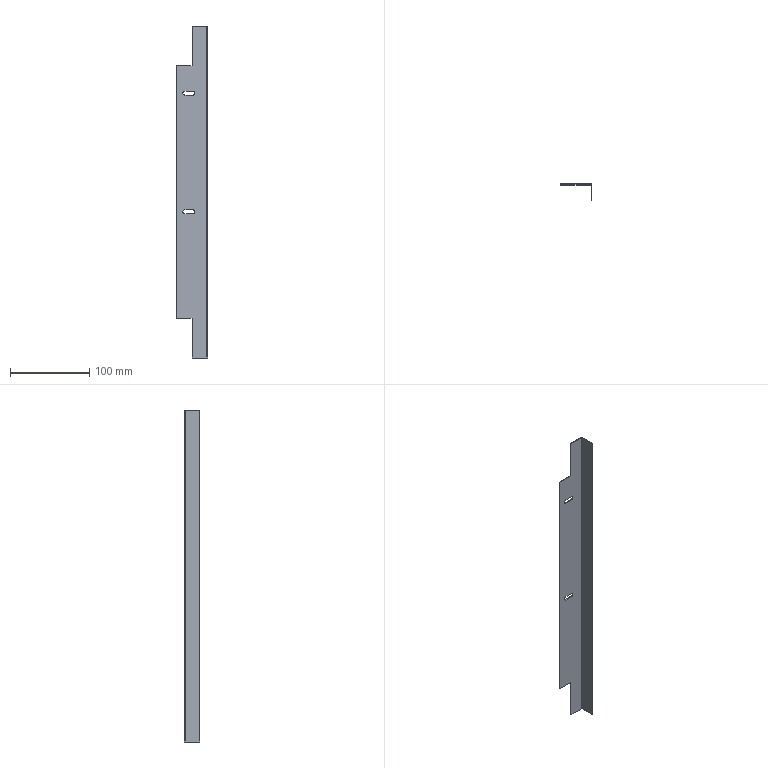Component | SolidWorks | CCQ-1.1-2UpperAngleIron-2 | 1 solid | 28 faces | box 40 x 20 x 420 mm | volume 22418 mm3 | plane 20 | cylinder 8 | commonest cylinder face diameters 5 x6 3.473 x1 1.473 x1 | material 304
STEP:
#1=COLOUR_RGB('',0.7922,0.8196,0.9333);
#2=FILL_AREA_STYLE_COLOUR('',#1);
#3=FILL_AREA_STYLE('',(#2));
#4=SURFACE_STYLE_FILL_AREA(#3);
#5=SURFACE_SIDE_STYLE('',(#4));
#6=SURFACE_STYLE_USAGE(.BOTH.,#5);
#7=PRESENTATION_STYLE_ASSIGNMENT((#6));
#8=CARTESIAN_POINT('',(0.2953,19.547,-8.819));
#9=VERTEX_POINT('',#8);
#10=CARTESIAN_POINT('',(0.3937,19.547,-8.72));
#11=VERTEX_POINT('',#10);
#12=CARTESIAN_POINT('',(0.3937,19.547,-8.819));
#13=DIRECTION('',(-0.,1.,0.));
#14=DIRECTION('',(-1.,0.,0.));
#15=AXIS2_PLACEMENT_3D('',#12,#13,#14);
#16=CIRCLE('',#15,0.09843);
#17=EDGE_CURVE('',#9,#11,#16,.T.);
#18=ORIENTED_EDGE('',*,*,#17,.F.);
#19=CARTESIAN_POINT('',(0.2953,19.587,-8.819));
#20=VERTEX_POINT('',#19);
#21=CARTESIAN_POINT('',(0.2953,19.193,-8.819));
#22=DIRECTION('',(-0.,1.,0.));
#23=VECTOR('',#22,39.37);
#24=LINE('',#21,#23);
#25=EDGE_CURVE('',#9,#20,#24,.T.);
#26=ORIENTED_EDGE('',*,*,#25,.T.);
#27=CARTESIAN_POINT('',(0.3937,19.587,-8.72));
#28=VERTEX_POINT('',#27);
#29=CARTESIAN_POINT('',(0.3937,19.587,-8.819));
#30=DIRECTION('',(-0.,1.,0.));
#31=DIRECTION('',(-1.,0.,0.));
#32=AXIS2_PLACEMENT_3D('',#29,#30,#31);
#33=CIRCLE('',#32,0.09843);
#34=EDGE_CURVE('',#20,#28,#33,.T.);
#35=ORIENTED_EDGE('',*,*,#34,.T.);
#36=CARTESIAN_POINT('',(0.3937,19.193,-8.72));
#37=DIRECTION('',(-0.,1.,0.));
#38=VECTOR('',#37,39.37);
#39=LINE('',#36,#38);
#40=EDGE_CURVE('',#11,#28,#39,.T.);
#41=ORIENTED_EDGE('',*,*,#40,.F.);
#42=EDGE_LOOP('',(#18,#26,#35,#41));
#43=FACE_OUTER_BOUND('',#42,.T.);
#44=CARTESIAN_POINT('',(0.3937,19.193,-8.819));
#45=DIRECTION('',(-0.,1.,0.));
#46=DIRECTION('',(-1.,0.,0.));
#47=AXIS2_PLACEMENT_3D('',#44,#45,#46);
#48=CYLINDRICAL_SURFACE('',#47,0.09843);
#49=ADVANCED_FACE('',(#43),#48,.F.);
#50=CARTESIAN_POINT('',(0.2953,19.547,-2.913));
#51=VERTEX_POINT('',#50);
#52=CARTESIAN_POINT('',(0.3937,19.547,-2.815));
#53=VERTEX_POINT('',#52);
#54=CARTESIAN_POINT('',(0.3937,19.547,-2.913));
#55=DIRECTION('',(-0.,1.,0.));
#56=DIRECTION('',(-1.,0.,0.));
#57=AXIS2_PLACEMENT_3D('',#54,#55,#56);
#58=CIRCLE('',#57,0.09843);
#59=EDGE_CURVE('',#51,#53,#58,.T.);
#60=ORIENTED_EDGE('',*,*,#59,.F.);
#61=CARTESIAN_POINT('',(0.2953,19.587,-2.913));
#62=VERTEX_POINT('',#61);
#63=CARTESIAN_POINT('',(0.2953,19.193,-2.913));
#64=DIRECTION('',(-0.,1.,0.));
#65=VECTOR('',#64,39.37);
#66=LINE('',#63,#65);
#67=EDGE_CURVE('',#51,#62,#66,.T.);
#68=ORIENTED_EDGE('',*,*,#67,.T.);
#69=CARTESIAN_POINT('',(0.3937,19.587,-2.815));
#70=VERTEX_POINT('',#69);
#71=CARTESIAN_POINT('',(0.3937,19.587,-2.913));
#72=DIRECTION('',(-0.,1.,0.));
#73=DIRECTION('',(-1.,0.,0.));
#74=AXIS2_PLACEMENT_3D('',#71,#72,#73);
#75=CIRCLE('',#74,0.09843);
#76=EDGE_CURVE('',#62,#70,#75,.T.);
#77=ORIENTED_EDGE('',*,*,#76,.T.);
#78=CARTESIAN_POINT('',(0.3937,19.193,-2.815));
#79=DIRECTION('',(-0.,1.,0.));
#80=VECTOR('',#79,39.37);
#81=LINE('',#78,#80);
#82=EDGE_CURVE('',#53,#70,#81,.T.);
#83=ORIENTED_EDGE('',*,*,#82,.F.);
#84=EDGE_LOOP('',(#60,#68,#77,#83));
#85=FACE_OUTER_BOUND('',#84,.T.);
#86=CARTESIAN_POINT('',(0.3937,19.193,-2.913));
#87=DIRECTION('',(-0.,1.,0.));
#88=DIRECTION('',(-1.,0.,0.));
#89=AXIS2_PLACEMENT_3D('',#86,#87,#88);
#90=CYLINDRICAL_SURFACE('',#89,0.09843);
#91=ADVANCED_FACE('',(#85),#90,.F.);
#92=CARTESIAN_POINT('',(1.535,19.518,0.4331));
#93=VERTEX_POINT('',#92);
#94=CARTESIAN_POINT('',(1.496,19.518,0.4331));
#95=VERTEX_POINT('',#94);
#96=CARTESIAN_POINT('',(1.535,19.518,0.4331));
#97=DIRECTION('',(-1.,-0.,0.));
#98=VECTOR('',#97,39.37);
#99=LINE('',#96,#98);
#100=EDGE_CURVE('',#93,#95,#99,.T.);
#101=ORIENTED_EDGE('',*,*,#100,.F.);
#102=CARTESIAN_POINT('',(1.467,19.587,0.4331));
#103=VERTEX_POINT('',#102);
#104=CARTESIAN_POINT('',(1.467,19.518,0.4331));
#105=DIRECTION('',(-0.,0.,-1.));
#106=DIRECTION('',(1.,0.,0.));
#107=AXIS2_PLACEMENT_3D('',#104,#105,#106);
#108=CIRCLE('',#107,0.06837);
#109=EDGE_CURVE('',#103,#93,#108,.T.);
#110=ORIENTED_EDGE('',*,*,#109,.F.);
#111=CARTESIAN_POINT('',(1.467,19.547,0.4331));
#112=VERTEX_POINT('',#111);
#113=CARTESIAN_POINT('',(1.467,19.547,0.4331));
#114=DIRECTION('',(0.,1.,0.));
#115=VECTOR('',#114,39.37);
#116=LINE('',#113,#115);
#117=EDGE_CURVE('',#112,#103,#116,.T.);
#118=ORIENTED_EDGE('',*,*,#117,.F.);
#119=CARTESIAN_POINT('',(1.467,19.518,0.4331));
#120=DIRECTION('',(-0.,0.,-1.));
#121=DIRECTION('',(1.,0.,0.));
#122=AXIS2_PLACEMENT_3D('',#119,#120,#121);
#123=CIRCLE('',#122,0.029);
#124=EDGE_CURVE('',#112,#95,#123,.T.);
#125=ORIENTED_EDGE('',*,*,#124,.T.);
#126=EDGE_LOOP('',(#101,#110,#118,#125));
#127=FACE_OUTER_BOUND('',#126,.T.);
#128=CARTESIAN_POINT('',(1.535,19.518,0.4331));
#129=DIRECTION('',(0.,-0.,1.));
#130=DIRECTION('',(1.,0.,-0.));
#131=AXIS2_PLACEMENT_3D('',#128,#129,#130);
#132=PLANE('',#131);
#133=ADVANCED_FACE('',(#127),#132,.T.);
#134=CARTESIAN_POINT('',(1.535,18.799,0.4331));
#135=VERTEX_POINT('',#134);
#136=CARTESIAN_POINT('',(1.535,19.587,0.4331));
#137=DIRECTION('',(0.,-1.,-0.));
#138=VECTOR('',#137,39.37);
#139=LINE('',#136,#138);
#140=EDGE_CURVE('',#93,#135,#139,.T.);
#141=ORIENTED_EDGE('',*,*,#140,.F.);
#142=ORIENTED_EDGE('',*,*,#100,.T.);
#143=CARTESIAN_POINT('',(1.496,18.799,0.4331));
#144=VERTEX_POINT('',#143);
#145=CARTESIAN_POINT('',(1.496,19.587,0.4331));
#146=DIRECTION('',(0.,-1.,-0.));
#147=VECTOR('',#146,39.37);
#148=LINE('',#145,#147);
#149=EDGE_CURVE('',#95,#144,#148,.T.);
#150=ORIENTED_EDGE('',*,*,#149,.T.);
#151=CARTESIAN_POINT('',(1.535,18.799,0.4331));
#152=DIRECTION('',(-1.,-0.,0.));
#153=VECTOR('',#152,39.37);
#154=LINE('',#151,#153);
#155=EDGE_CURVE('',#135,#144,#154,.T.);
#156=ORIENTED_EDGE('',*,*,#155,.F.);
#157=EDGE_LOOP('',(#141,#142,#150,#156));
#158=FACE_OUTER_BOUND('',#157,.T.);
#159=CARTESIAN_POINT('',(1.467,19.547,0.4331));
#160=DIRECTION('',(0.,-0.,1.));
#161=DIRECTION('',(1.,0.,-0.));
#162=AXIS2_PLACEMENT_3D('',#159,#160,#161);
#163=PLANE('',#162);
#164=ADVANCED_FACE('',(#158),#163,.T.);
#165=CARTESIAN_POINT('',(1.467,19.587,-16.102));
#166=VERTEX_POINT('',#165);
#167=CARTESIAN_POINT('',(1.467,19.547,-16.102));
#168=VERTEX_POINT('',#167);
#169=CARTESIAN_POINT('',(1.467,19.587,-16.102));
#170=DIRECTION('',(-0.,-1.,-0.));
#171=VECTOR('',#170,39.37);
#172=LINE('',#169,#171);
#173=EDGE_CURVE('',#166,#168,#172,.T.);
#174=ORIENTED_EDGE('',*,*,#173,.F.);
#175=CARTESIAN_POINT('',(1.535,19.518,-16.102));
#176=VERTEX_POINT('',#175);
#177=CARTESIAN_POINT('',(1.467,19.518,-16.102));
#178=DIRECTION('',(-0.,0.,-1.));
#179=DIRECTION('',(1.,0.,0.));
#180=AXIS2_PLACEMENT_3D('',#177,#178,#179);
#181=CIRCLE('',#180,0.06837);
#182=EDGE_CURVE('',#166,#176,#181,.T.);
#183=ORIENTED_EDGE('',*,*,#182,.T.);
#184=CARTESIAN_POINT('',(1.496,19.518,-16.102));
#185=VERTEX_POINT('',#184);
#186=CARTESIAN_POINT('',(1.496,19.518,-16.102));
#187=DIRECTION('',(1.,0.,-0.));
#188=VECTOR('',#187,39.37);
#189=LINE('',#186,#188);
#190=EDGE_CURVE('',#185,#176,#189,.T.);
#191=ORIENTED_EDGE('',*,*,#190,.F.);
#192=CARTESIAN_POINT('',(1.467,19.518,-16.102));
#193=DIRECTION('',(-0.,0.,-1.));
#194=DIRECTION('',(1.,0.,0.));
#195=AXIS2_PLACEMENT_3D('',#192,#193,#194);
#196=CIRCLE('',#195,0.029);
#197=EDGE_CURVE('',#168,#185,#196,.T.);
#198=ORIENTED_EDGE('',*,*,#197,.F.);
#199=EDGE_LOOP('',(#174,#183,#191,#198));
#200=FACE_OUTER_BOUND('',#199,.T.);
#201=CARTESIAN_POINT('',(1.467,19.587,-16.102));
#202=DIRECTION('',(-0.,0.,-1.));
#203=DIRECTION('',(-1.,-0.,0.));
#204=AXIS2_PLACEMENT_3D('',#201,#202,#203);
#205=PLANE('',#204);
#206=ADVANCED_FACE('',(#200),#205,.T.);
#207=CARTESIAN_POINT('',(0.748,19.547,-16.102));
#208=VERTEX_POINT('',#207);
#209=CARTESIAN_POINT('',(0.748,19.587,-16.102));
#210=VERTEX_POINT('',#209);
#211=CARTESIAN_POINT('',(0.748,19.193,-16.102));
#212=DIRECTION('',(-0.,1.,0.));
#213=VECTOR('',#212,39.37);
#214=LINE('',#211,#213);
#215=EDGE_CURVE('',#208,#210,#214,.T.);
#216=ORIENTED_EDGE('',*,*,#215,.T.);
#217=CARTESIAN_POINT('',(-0.03937,19.587,-16.102));
#218=DIRECTION('',(1.,0.,-0.));
#219=VECTOR('',#218,39.37);
#220=LINE('',#217,#219);
#221=EDGE_CURVE('',#210,#166,#220,.T.);
#222=ORIENTED_EDGE('',*,*,#221,.T.);
#223=ORIENTED_EDGE('',*,*,#173,.T.);
#224=CARTESIAN_POINT('',(-0.03937,19.547,-16.102));
#225=DIRECTION('',(1.,0.,-0.));
#226=VECTOR('',#225,39.37);
#227=LINE('',#224,#226);
#228=EDGE_CURVE('',#208,#168,#227,.T.);
#229=ORIENTED_EDGE('',*,*,#228,.F.);
#230=EDGE_LOOP('',(#216,#222,#223,#229));
#231=FACE_OUTER_BOUND('',#230,.T.);
#232=CARTESIAN_POINT('',(1.496,19.518,-16.102));
#233=DIRECTION('',(-0.,0.,-1.));
#234=DIRECTION('',(-1.,-0.,0.));
#235=AXIS2_PLACEMENT_3D('',#232,#233,#234);
#236=PLANE('',#235);
#237=ADVANCED_FACE('',(#231),#236,.T.);
#238=CARTESIAN_POINT('',(1.496,18.799,-16.102));
#239=VERTEX_POINT('',#238);
#240=CARTESIAN_POINT('',(1.496,19.587,-16.102));
#241=DIRECTION('',(0.,-1.,-0.));
#242=VECTOR('',#241,39.37);
#243=LINE('',#240,#242);
#244=EDGE_CURVE('',#185,#239,#243,.T.);
#245=ORIENTED_EDGE('',*,*,#244,.T.);
#246=CARTESIAN_POINT('',(1.496,18.799,0.4331));
#247=DIRECTION('',(-0.,0.,-1.));
#248=VECTOR('',#247,39.37);
#249=LINE('',#246,#248);
#250=EDGE_CURVE('',#144,#239,#249,.T.);
#251=ORIENTED_EDGE('',*,*,#250,.F.);
#252=ORIENTED_EDGE('',*,*,#149,.F.);
#253=CARTESIAN_POINT('',(1.496,19.518,0.4331));
#254=DIRECTION('',(-0.,0.,-1.));
#255=VECTOR('',#254,39.37);
#256=LINE('',#253,#255);
#257=EDGE_CURVE('',#95,#185,#256,.T.);
#258=ORIENTED_EDGE('',*,*,#257,.T.);
#259=EDGE_LOOP('',(#245,#251,#252,#258));
#260=FACE_OUTER_BOUND('',#259,.T.);
#261=CARTESIAN_POINT('',(1.496,19.587,0.4331));
#262=DIRECTION('',(1.,0.,-0.));
#263=DIRECTION('',(-0.,0.,-1.));
#264=AXIS2_PLACEMENT_3D('',#261,#262,#263);
#265=PLANE('',#264);
#266=ADVANCED_FACE('',(#260),#265,.F.);
#267=CARTESIAN_POINT('',(1.535,18.799,-16.102));
#268=VERTEX_POINT('',#267);
#269=CARTESIAN_POINT('',(1.535,18.799,-16.102));
#270=DIRECTION('',(-1.,-0.,0.));
#271=VECTOR('',#270,39.37);
#272=LINE('',#269,#271);
#273=EDGE_CURVE('',#268,#239,#272,.T.);
#274=ORIENTED_EDGE('',*,*,#273,.F.);
#275=CARTESIAN_POINT('',(1.535,18.799,0.4331));
#276=DIRECTION('',(-0.,0.,-1.));
#277=VECTOR('',#276,39.37);
#278=LINE('',#275,#277);
#279=EDGE_CURVE('',#135,#268,#278,.T.);
#280=ORIENTED_EDGE('',*,*,#279,.F.);
#281=ORIENTED_EDGE('',*,*,#155,.T.);
#282=ORIENTED_EDGE('',*,*,#250,.T.);
#283=EDGE_LOOP('',(#274,#280,#281,#282));
#284=FACE_OUTER_BOUND('',#283,.T.);
#285=CARTESIAN_POINT('',(1.535,18.799,0.4331));
#286=DIRECTION('',(0.,-1.,-0.));
#287=DIRECTION('',(1.,0.,-0.));
#288=AXIS2_PLACEMENT_3D('',#285,#286,#287);
#289=PLANE('',#288);
#290=ADVANCED_FACE('',(#284),#289,.T.);
#291=CARTESIAN_POINT('',(1.535,19.587,-16.102));
#292=DIRECTION('',(0.,-1.,-0.));
#293=VECTOR('',#292,39.37);
#294=LINE('',#291,#293);
#295=EDGE_CURVE('',#176,#268,#294,.T.);
#296=ORIENTED_EDGE('',*,*,#295,.F.);
#297=CARTESIAN_POINT('',(1.535,19.518,0.4331));
#298=DIRECTION('',(-0.,0.,-1.));
#299=VECTOR('',#298,39.37);
#300=LINE('',#297,#299);
#301=EDGE_CURVE('',#93,#176,#300,.T.);
#302=ORIENTED_EDGE('',*,*,#301,.F.);
#303=ORIENTED_EDGE('',*,*,#140,.T.);
#304=ORIENTED_EDGE('',*,*,#279,.T.);
#305=EDGE_LOOP('',(#296,#302,#303,#304));
#306=FACE_OUTER_BOUND('',#305,.T.);
#307=CARTESIAN_POINT('',(1.535,19.587,0.4331));
#308=DIRECTION('',(1.,0.,-0.));
#309=DIRECTION('',(-0.,0.,-1.));
#310=AXIS2_PLACEMENT_3D('',#307,#308,#309);
#311=PLANE('',#310);
#312=ADVANCED_FACE('',(#306),#311,.T.);
#313=ORIENTED_EDGE('',*,*,#182,.F.);
#314=CARTESIAN_POINT('',(1.467,19.587,0.4331));
#315=DIRECTION('',(-0.,0.,-1.));
#316=VECTOR('',#315,39.37);
#317=LINE('',#314,#316);
#318=EDGE_CURVE('',#103,#166,#317,.T.);
#319=ORIENTED_EDGE('',*,*,#318,.F.);
#320=ORIENTED_EDGE('',*,*,#109,.T.);
#321=ORIENTED_EDGE('',*,*,#301,.T.);
#322=EDGE_LOOP('',(#313,#319,#320,#321));
#323=FACE_OUTER_BOUND('',#322,.T.);
#324=CARTESIAN_POINT('',(1.467,19.518,0.4331));
#325=DIRECTION('',(-0.,0.,-1.));
#326=DIRECTION('',(-1.,0.,0.));
#327=AXIS2_PLACEMENT_3D('',#324,#325,#326);
#328=CYLINDRICAL_SURFACE('',#327,0.06837);
#329=ADVANCED_FACE('',(#323),#328,.T.);
#330=CARTESIAN_POINT('',(0.7874,19.587,-8.72));
#331=VERTEX_POINT('',#330);
#332=CARTESIAN_POINT('',(0.7874,19.587,-8.917));
#333=VERTEX_POINT('',#332);
#334=CARTESIAN_POINT('',(0.7874,19.587,-8.819));
#335=DIRECTION('',(-0.,1.,0.));
#336=DIRECTION('',(-1.,0.,0.));
#337=AXIS2_PLACEMENT_3D('',#334,#335,#336);
#338=CIRCLE('',#337,0.09843);
#339=EDGE_CURVE('',#331,#333,#338,.T.);
#340=ORIENTED_EDGE('',*,*,#339,.F.);
#341=CARTESIAN_POINT('',(0.7874,19.587,-8.72));
#342=DIRECTION('',(1.,0.,-0.));
#343=VECTOR('',#342,39.37);
#344=LINE('',#341,#343);
#345=EDGE_CURVE('',#28,#331,#344,.T.);
#346=ORIENTED_EDGE('',*,*,#345,.F.);
#347=ORIENTED_EDGE('',*,*,#34,.F.);
#348=CARTESIAN_POINT('',(0.3937,19.587,-8.917));
#349=VERTEX_POINT('',#348);
#350=CARTESIAN_POINT('',(0.3937,19.587,-8.819));
#351=DIRECTION('',(-0.,1.,0.));
#352=DIRECTION('',(-1.,0.,0.));
#353=AXIS2_PLACEMENT_3D('',#350,#351,#352);
#354=CIRCLE('',#353,0.09843);
#355=EDGE_CURVE('',#349,#20,#354,.T.);
#356=ORIENTED_EDGE('',*,*,#355,.F.);
#357=CARTESIAN_POINT('',(0.7874,19.587,-8.917));
#358=DIRECTION('',(-1.,-0.,0.));
#359=VECTOR('',#358,39.37);
#360=LINE('',#357,#359);
#361=EDGE_CURVE('',#333,#349,#360,.T.);
#362=ORIENTED_EDGE('',*,*,#361,.F.);
#363=EDGE_LOOP('',(#340,#346,#347,#356,#362));
#364=FACE_BOUND('',#363,.T.);
#365=CARTESIAN_POINT('',(0.7874,19.587,-2.815));
#366=VERTEX_POINT('',#365);
#367=CARTESIAN_POINT('',(0.7874,19.587,-3.012));
#368=VERTEX_POINT('',#367);
#369=CARTESIAN_POINT('',(0.7874,19.587,-2.913));
#370=DIRECTION('',(-0.,1.,0.));
#371=DIRECTION('',(-1.,0.,0.));
#372=AXIS2_PLACEMENT_3D('',#369,#370,#371);
#373=CIRCLE('',#372,0.09843);
#374=EDGE_CURVE('',#366,#368,#373,.T.);
#375=ORIENTED_EDGE('',*,*,#374,.F.);
#376=CARTESIAN_POINT('',(0.7874,19.587,-2.815));
#377=DIRECTION('',(1.,0.,-0.));
#378=VECTOR('',#377,39.37);
#379=LINE('',#376,#378);
#380=EDGE_CURVE('',#70,#366,#379,.T.);
#381=ORIENTED_EDGE('',*,*,#380,.F.);
#382=ORIENTED_EDGE('',*,*,#76,.F.);
#383=CARTESIAN_POINT('',(0.3937,19.587,-3.012));
#384=VERTEX_POINT('',#383);
#385=CARTESIAN_POINT('',(0.3937,19.587,-2.913));
#386=DIRECTION('',(-0.,1.,0.));
#387=DIRECTION('',(-1.,0.,0.));
#388=AXIS2_PLACEMENT_3D('',#385,#386,#387);
#389=CIRCLE('',#388,0.09843);
#390=EDGE_CURVE('',#384,#62,#389,.T.);
#391=ORIENTED_EDGE('',*,*,#390,.F.);
#392=CARTESIAN_POINT('',(0.7874,19.587,-3.012));
#393=DIRECTION('',(-1.,-0.,0.));
#394=VECTOR('',#393,39.37);
#395=LINE('',#392,#394);
#396=EDGE_CURVE('',#368,#384,#395,.T.);
#397=ORIENTED_EDGE('',*,*,#396,.F.);
#398=EDGE_LOOP('',(#375,#381,#382,#391,#397));
#399=FACE_BOUND('',#398,.T.);
#400=CARTESIAN_POINT('',(0.748,19.587,0.4331));
#401=VERTEX_POINT('',#400);
#402=CARTESIAN_POINT('',(0.748,19.587,-1.535));
#403=VERTEX_POINT('',#402);
#404=CARTESIAN_POINT('',(0.748,19.587,0.4331));
#405=DIRECTION('',(-0.,0.,-1.));
#406=VECTOR('',#405,39.37);
#407=LINE('',#404,#406);
#408=EDGE_CURVE('',#401,#403,#407,.T.);
#409=ORIENTED_EDGE('',*,*,#408,.F.);
#410=CARTESIAN_POINT('',(-0.03937,19.587,0.4331));
#411=DIRECTION('',(1.,0.,-0.));
#412=VECTOR('',#411,39.37);
#413=LINE('',#410,#412);
#414=EDGE_CURVE('',#401,#103,#413,.T.);
#415=ORIENTED_EDGE('',*,*,#414,.T.);
#416=ORIENTED_EDGE('',*,*,#318,.T.);
#417=ORIENTED_EDGE('',*,*,#221,.F.);
#418=CARTESIAN_POINT('',(0.748,19.587,-14.134));
#419=VERTEX_POINT('',#418);
#420=CARTESIAN_POINT('',(0.748,19.587,-16.102));
#421=DIRECTION('',(-0.,0.,-1.));
#422=VECTOR('',#421,39.37);
#423=LINE('',#420,#422);
#424=EDGE_CURVE('',#419,#210,#423,.T.);
#425=ORIENTED_EDGE('',*,*,#424,.F.);
#426=CARTESIAN_POINT('',(-0.03937,19.587,-14.134));
#427=VERTEX_POINT('',#426);
#428=CARTESIAN_POINT('',(0.748,19.587,-14.134));
#429=DIRECTION('',(1.,0.,-0.));
#430=VECTOR('',#429,39.37);
#431=LINE('',#428,#430);
#432=EDGE_CURVE('',#427,#419,#431,.T.);
#433=ORIENTED_EDGE('',*,*,#432,.F.);
#434=CARTESIAN_POINT('',(-0.03937,19.587,-1.535));
#435=VERTEX_POINT('',#434);
#436=CARTESIAN_POINT('',(-0.03937,19.587,0.4331));
#437=DIRECTION('',(-0.,0.,-1.));
#438=VECTOR('',#437,39.37);
#439=LINE('',#436,#438);
#440=EDGE_CURVE('',#435,#427,#439,.T.);
#441=ORIENTED_EDGE('',*,*,#440,.F.);
#442=CARTESIAN_POINT('',(0.748,19.587,-1.535));
#443=DIRECTION('',(-1.,-0.,0.));
#444=VECTOR('',#443,39.37);
#445=LINE('',#442,#444);
#446=EDGE_CURVE('',#403,#435,#445,.T.);
#447=ORIENTED_EDGE('',*,*,#446,.F.);
#448=EDGE_LOOP('',(#409,#415,#416,#417,#425,#433,#441,#447));
#449=FACE_OUTER_BOUND('',#448,.T.);
#450=CARTESIAN_POINT('',(-0.03937,19.587,0.4331));
#451=DIRECTION('',(-0.,1.,0.));
#452=DIRECTION('',(-1.,-0.,0.));
#453=AXIS2_PLACEMENT_3D('',#450,#451,#452);
#454=PLANE('',#453);
#455=ADVANCED_FACE('',(#364,#399,#449),#454,.T.);
#456=CARTESIAN_POINT('',(-0.03937,19.547,-1.535));
#457=VERTEX_POINT('',#456);
#458=CARTESIAN_POINT('',(-0.03937,19.193,-1.535));
#459=DIRECTION('',(-0.,1.,0.));
#460=VECTOR('',#459,39.37);
#461=LINE('',#458,#460);
#462=EDGE_CURVE('',#457,#435,#461,.T.);
#463=ORIENTED_EDGE('',*,*,#462,.T.);
#464=ORIENTED_EDGE('',*,*,#440,.T.);
#465=CARTESIAN_POINT('',(-0.03937,19.547,-14.134));
#466=VERTEX_POINT('',#465);
#467=CARTESIAN_POINT('',(-0.03937,19.193,-14.134));
#468=DIRECTION('',(-0.,1.,0.));
#469=VECTOR('',#468,39.37);
#470=LINE('',#467,#469);
#471=EDGE_CURVE('',#466,#427,#470,.T.);
#472=ORIENTED_EDGE('',*,*,#471,.F.);
#473=CARTESIAN_POINT('',(-0.03937,19.547,0.4331));
#474=DIRECTION('',(-0.,0.,-1.));
#475=VECTOR('',#474,39.37);
#476=LINE('',#473,#475);
#477=EDGE_CURVE('',#457,#466,#476,.T.);
#478=ORIENTED_EDGE('',*,*,#477,.F.);
#479=EDGE_LOOP('',(#463,#464,#472,#478));
#480=FACE_OUTER_BOUND('',#479,.T.);
#481=CARTESIAN_POINT('',(-0.03937,19.547,0.4331));
#482=DIRECTION('',(-1.,-0.,0.));
#483=DIRECTION('',(0.,-0.,1.));
#484=AXIS2_PLACEMENT_3D('',#481,#482,#483);
#485=PLANE('',#484);
#486=ADVANCED_FACE('',(#480),#485,.T.);
#487=CARTESIAN_POINT('',(0.7874,19.547,-8.72));
#488=VERTEX_POINT('',#487);
#489=CARTESIAN_POINT('',(-0.03937,19.547,-8.72));
#490=DIRECTION('',(1.,0.,-0.));
#491=VECTOR('',#490,39.37);
#492=LINE('',#489,#491);
#493=EDGE_CURVE('',#11,#488,#492,.T.);
#494=ORIENTED_EDGE('',*,*,#493,.T.);
#495=CARTESIAN_POINT('',(0.7874,19.547,-8.917));
#496=VERTEX_POINT('',#495);
#497=CARTESIAN_POINT('',(0.7874,19.547,-8.819));
#498=DIRECTION('',(-0.,1.,0.));
#499=DIRECTION('',(-1.,0.,0.));
#500=AXIS2_PLACEMENT_3D('',#497,#498,#499);
#501=CIRCLE('',#500,0.09843);
#502=EDGE_CURVE('',#488,#496,#501,.T.);
#503=ORIENTED_EDGE('',*,*,#502,.T.);
#504=CARTESIAN_POINT('',(0.3937,19.547,-8.917));
#505=VERTEX_POINT('',#504);
#506=CARTESIAN_POINT('',(-0.03937,19.547,-8.917));
#507=DIRECTION('',(-1.,-0.,0.));
#508=VECTOR('',#507,39.37);
#509=LINE('',#506,#508);
#510=EDGE_CURVE('',#496,#505,#509,.T.);
#511=ORIENTED_EDGE('',*,*,#510,.T.);
#512=CARTESIAN_POINT('',(0.3937,19.547,-8.819));
#513=DIRECTION('',(-0.,1.,0.));
#514=DIRECTION('',(-1.,0.,0.));
#515=AXIS2_PLACEMENT_3D('',#512,#513,#514);
#516=CIRCLE('',#515,0.09843);
#517=EDGE_CURVE('',#505,#9,#516,.T.);
#518=ORIENTED_EDGE('',*,*,#517,.T.);
#519=ORIENTED_EDGE('',*,*,#17,.T.);
#520=EDGE_LOOP('',(#494,#503,#511,#518,#519));
#521=FACE_BOUND('',#520,.T.);
#522=CARTESIAN_POINT('',(0.7874,19.547,-2.815));
#523=VERTEX_POINT('',#522);
#524=CARTESIAN_POINT('',(-0.03937,19.547,-2.815));
#525=DIRECTION('',(1.,0.,-0.));
#526=VECTOR('',#525,39.37);
#527=LINE('',#524,#526);
#528=EDGE_CURVE('',#53,#523,#527,.T.);
#529=ORIENTED_EDGE('',*,*,#528,.T.);
#530=CARTESIAN_POINT('',(0.7874,19.547,-3.012));
#531=VERTEX_POINT('',#530);
#532=CARTESIAN_POINT('',(0.7874,19.547,-2.913));
#533=DIRECTION('',(-0.,1.,0.));
#534=DIRECTION('',(-1.,0.,0.));
#535=AXIS2_PLACEMENT_3D('',#532,#533,#534);
#536=CIRCLE('',#535,0.09843);
#537=EDGE_CURVE('',#523,#531,#536,.T.);
#538=ORIENTED_EDGE('',*,*,#537,.T.);
#539=CARTESIAN_POINT('',(0.3937,19.547,-3.012));
#540=VERTEX_POINT('',#539);
#541=CARTESIAN_POINT('',(-0.03937,19.547,-3.012));
#542=DIRECTION('',(-1.,-0.,0.));
#543=VECTOR('',#542,39.37);
#544=LINE('',#541,#543);
#545=EDGE_CURVE('',#531,#540,#544,.T.);
#546=ORIENTED_EDGE('',*,*,#545,.T.);
#547=CARTESIAN_POINT('',(0.3937,19.547,-2.913));
#548=DIRECTION('',(-0.,1.,0.));
#549=DIRECTION('',(-1.,0.,0.));
#550=AXIS2_PLACEMENT_3D('',#547,#548,#549);
#551=CIRCLE('',#550,0.09843);
#552=EDGE_CURVE('',#540,#51,#551,.T.);
#553=ORIENTED_EDGE('',*,*,#552,.T.);
#554=ORIENTED_EDGE('',*,*,#59,.T.);
#555=EDGE_LOOP('',(#529,#538,#546,#553,#554));
#556=FACE_BOUND('',#555,.T.);
#557=CARTESIAN_POINT('',(0.748,19.547,0.4331));
#558=VERTEX_POINT('',#557);
#559=CARTESIAN_POINT('',(-0.03937,19.547,0.4331));
#560=DIRECTION('',(1.,0.,-0.));
#561=VECTOR('',#560,39.37);
#562=LINE('',#559,#561);
#563=EDGE_CURVE('',#558,#112,#562,.T.);
#564=ORIENTED_EDGE('',*,*,#563,.F.);
#565=CARTESIAN_POINT('',(0.748,19.547,-1.535));
#566=VERTEX_POINT('',#565);
#567=CARTESIAN_POINT('',(0.748,19.547,0.4331));
#568=DIRECTION('',(-0.,0.,-1.));
#569=VECTOR('',#568,39.37);
#570=LINE('',#567,#569);
#571=EDGE_CURVE('',#558,#566,#570,.T.);
#572=ORIENTED_EDGE('',*,*,#571,.T.);
#573=CARTESIAN_POINT('',(-0.03937,19.547,-1.535));
#574=DIRECTION('',(-1.,-0.,0.));
#575=VECTOR('',#574,39.37);
#576=LINE('',#573,#575);
#577=EDGE_CURVE('',#566,#457,#576,.T.);
#578=ORIENTED_EDGE('',*,*,#577,.T.);
#579=ORIENTED_EDGE('',*,*,#477,.T.);
#580=CARTESIAN_POINT('',(0.748,19.547,-14.134));
#581=VERTEX_POINT('',#580);
#582=CARTESIAN_POINT('',(-0.03937,19.547,-14.134));
#583=DIRECTION('',(1.,0.,-0.));
#584=VECTOR('',#583,39.37);
#585=LINE('',#582,#584);
#586=EDGE_CURVE('',#466,#581,#585,.T.);
#587=ORIENTED_EDGE('',*,*,#586,.T.);
#588=CARTESIAN_POINT('',(0.748,19.547,0.4331));
#589=DIRECTION('',(-0.,0.,-1.));
#590=VECTOR('',#589,39.37);
#591=LINE('',#588,#590);
#592=EDGE_CURVE('',#581,#208,#591,.T.);
#593=ORIENTED_EDGE('',*,*,#592,.T.);
#594=ORIENTED_EDGE('',*,*,#228,.T.);
#595=CARTESIAN_POINT('',(1.467,19.547,0.4331));
#596=DIRECTION('',(-0.,0.,-1.));
#597=VECTOR('',#596,39.37);
#598=LINE('',#595,#597);
#599=EDGE_CURVE('',#112,#168,#598,.T.);
#600=ORIENTED_EDGE('',*,*,#599,.F.);
#601=EDGE_LOOP('',(#564,#572,#578,#579,#587,#593,#594,#600));
#602=FACE_OUTER_BOUND('',#601,.T.);
#603=CARTESIAN_POINT('',(-0.03937,19.547,0.4331));
#604=DIRECTION('',(-0.,1.,0.));
#605=DIRECTION('',(-1.,-0.,0.));
#606=AXIS2_PLACEMENT_3D('',#603,#604,#605);
#607=PLANE('',#606);
#608=ADVANCED_FACE('',(#521,#556,#602),#607,.F.);
#609=ORIENTED_EDGE('',*,*,#197,.T.);
#610=ORIENTED_EDGE('',*,*,#257,.F.);
#611=ORIENTED_EDGE('',*,*,#124,.F.);
#612=ORIENTED_EDGE('',*,*,#599,.T.);
#613=EDGE_LOOP('',(#609,#610,#611,#612));
#614=FACE_OUTER_BOUND('',#613,.T.);
#615=CARTESIAN_POINT('',(1.467,19.518,0.4331));
#616=DIRECTION('',(-0.,0.,-1.));
#617=DIRECTION('',(-1.,0.,0.));
#618=AXIS2_PLACEMENT_3D('',#615,#616,#617);
#619=CYLINDRICAL_SURFACE('',#618,0.029);
#620=ADVANCED_FACE('',(#614),#619,.F.);
#621=CARTESIAN_POINT('',(0.748,19.518,0.4331));
#622=DIRECTION('',(-0.,1.,0.));
#623=VECTOR('',#622,39.37);
#624=LINE('',#621,#623);
#625=EDGE_CURVE('',#558,#401,#624,.T.);
#626=ORIENTED_EDGE('',*,*,#625,.F.);
#627=ORIENTED_EDGE('',*,*,#563,.T.);
#628=ORIENTED_EDGE('',*,*,#117,.T.);
#629=ORIENTED_EDGE('',*,*,#414,.F.);
#630=EDGE_LOOP('',(#626,#627,#628,#629));
#631=FACE_OUTER_BOUND('',#630,.T.);
#632=CARTESIAN_POINT('',(1.467,19.518,0.4331));
#633=DIRECTION('',(0.,-0.,1.));
#634=DIRECTION('',(1.,0.,-0.));
#635=AXIS2_PLACEMENT_3D('',#632,#633,#634);
#636=PLANE('',#635);
#637=ADVANCED_FACE('',(#631),#636,.T.);
#638=ORIENTED_EDGE('',*,*,#244,.F.);
#639=ORIENTED_EDGE('',*,*,#190,.T.);
#640=ORIENTED_EDGE('',*,*,#295,.T.);
#641=ORIENTED_EDGE('',*,*,#273,.T.);
#642=EDGE_LOOP('',(#638,#639,#640,#641));
#643=FACE_OUTER_BOUND('',#642,.T.);
#644=CARTESIAN_POINT('',(1.467,19.518,-16.102));
#645=DIRECTION('',(0.,-0.,1.));
#646=DIRECTION('',(1.,0.,-0.));
#647=AXIS2_PLACEMENT_3D('',#644,#645,#646);
#648=PLANE('',#647);
#649=ADVANCED_FACE('',(#643),#648,.F.);
#650=CARTESIAN_POINT('',(0.748,19.193,-14.134));
#651=DIRECTION('',(-0.,1.,0.));
#652=VECTOR('',#651,39.37);
#653=LINE('',#650,#652);
#654=EDGE_CURVE('',#581,#419,#653,.T.);
#655=ORIENTED_EDGE('',*,*,#654,.T.);
#656=ORIENTED_EDGE('',*,*,#424,.T.);
#657=ORIENTED_EDGE('',*,*,#215,.F.);
#658=ORIENTED_EDGE('',*,*,#592,.F.);
#659=EDGE_LOOP('',(#655,#656,#657,#658));
#660=FACE_OUTER_BOUND('',#659,.T.);
#661=CARTESIAN_POINT('',(0.748,19.193,-16.102));
#662=DIRECTION('',(1.,0.,-0.));
#663=DIRECTION('',(-0.,0.,-1.));
#664=AXIS2_PLACEMENT_3D('',#661,#662,#663);
#665=PLANE('',#664);
#666=ADVANCED_FACE('',(#660),#665,.F.);
#667=ORIENTED_EDGE('',*,*,#471,.T.);
#668=ORIENTED_EDGE('',*,*,#432,.T.);
#669=ORIENTED_EDGE('',*,*,#654,.F.);
#670=ORIENTED_EDGE('',*,*,#586,.F.);
#671=EDGE_LOOP('',(#667,#668,#669,#670));
#672=FACE_OUTER_BOUND('',#671,.T.);
#673=CARTESIAN_POINT('',(0.748,19.193,-14.134));
#674=DIRECTION('',(0.,-0.,1.));
#675=DIRECTION('',(1.,0.,-0.));
#676=AXIS2_PLACEMENT_3D('',#673,#674,#675);
#677=PLANE('',#676);
#678=ADVANCED_FACE('',(#672),#677,.F.);
#679=CARTESIAN_POINT('',(0.748,19.193,-1.535));
#680=DIRECTION('',(-0.,1.,0.));
#681=VECTOR('',#680,39.37);
#682=LINE('',#679,#681);
#683=EDGE_CURVE('',#566,#403,#682,.T.);
#684=ORIENTED_EDGE('',*,*,#683,.T.);
#685=ORIENTED_EDGE('',*,*,#446,.T.);
#686=ORIENTED_EDGE('',*,*,#462,.F.);
#687=ORIENTED_EDGE('',*,*,#577,.F.);
#688=EDGE_LOOP('',(#684,#685,#686,#687));
#689=FACE_OUTER_BOUND('',#688,.T.);
#690=CARTESIAN_POINT('',(0.748,19.193,-1.535));
#691=DIRECTION('',(-0.,0.,-1.));
#692=DIRECTION('',(-1.,-0.,0.));
#693=AXIS2_PLACEMENT_3D('',#690,#691,#692);
#694=PLANE('',#693);
#695=ADVANCED_FACE('',(#689),#694,.F.);
#696=ORIENTED_EDGE('',*,*,#625,.T.);
#697=ORIENTED_EDGE('',*,*,#408,.T.);
#698=ORIENTED_EDGE('',*,*,#683,.F.);
#699=ORIENTED_EDGE('',*,*,#571,.F.);
#700=EDGE_LOOP('',(#696,#697,#698,#699));
#701=FACE_OUTER_BOUND('',#700,.T.);
#702=CARTESIAN_POINT('',(0.748,19.193,0.4331));
#703=DIRECTION('',(1.,0.,-0.));
#704=DIRECTION('',(-0.,0.,-1.));
#705=AXIS2_PLACEMENT_3D('',#702,#703,#704);
#706=PLANE('',#705);
#707=ADVANCED_FACE('',(#701),#706,.F.);
#708=CARTESIAN_POINT('',(0.7874,19.193,-2.815));
#709=DIRECTION('',(-0.,1.,0.));
#710=VECTOR('',#709,39.37);
#711=LINE('',#708,#710);
#712=EDGE_CURVE('',#523,#366,#711,.T.);
#713=ORIENTED_EDGE('',*,*,#712,.T.);
#714=ORIENTED_EDGE('',*,*,#374,.T.);
#715=CARTESIAN_POINT('',(0.7874,19.193,-3.012));
#716=DIRECTION('',(-0.,1.,0.));
#717=VECTOR('',#716,39.37);
#718=LINE('',#715,#717);
#719=EDGE_CURVE('',#531,#368,#718,.T.);
#720=ORIENTED_EDGE('',*,*,#719,.F.);
#721=ORIENTED_EDGE('',*,*,#537,.F.);
#722=EDGE_LOOP('',(#713,#714,#720,#721));
#723=FACE_OUTER_BOUND('',#722,.T.);
#724=CARTESIAN_POINT('',(0.7874,19.193,-2.913));
#725=DIRECTION('',(-0.,1.,0.));
#726=DIRECTION('',(-1.,0.,0.));
#727=AXIS2_PLACEMENT_3D('',#724,#725,#726);
#728=CYLINDRICAL_SURFACE('',#727,0.09843);
#729=ADVANCED_FACE('',(#723),#728,.F.);
#730=ORIENTED_EDGE('',*,*,#82,.T.);
#731=ORIENTED_EDGE('',*,*,#380,.T.);
#732=ORIENTED_EDGE('',*,*,#712,.F.);
#733=ORIENTED_EDGE('',*,*,#528,.F.);
#734=EDGE_LOOP('',(#730,#731,#732,#733));
#735=FACE_OUTER_BOUND('',#734,.T.);
#736=CARTESIAN_POINT('',(0.7874,19.193,-2.815));
#737=DIRECTION('',(0.,-0.,1.));
#738=DIRECTION('',(1.,0.,-0.));
#739=AXIS2_PLACEMENT_3D('',#736,#737,#738);
#740=PLANE('',#739);
#741=ADVANCED_FACE('',(#735),#740,.F.);
#742=ORIENTED_EDGE('',*,*,#67,.F.);
#743=ORIENTED_EDGE('',*,*,#552,.F.);
#744=CARTESIAN_POINT('',(0.3937,19.193,-3.012));
#745=DIRECTION('',(-0.,1.,0.));
#746=VECTOR('',#745,39.37);
#747=LINE('',#744,#746);
#748=EDGE_CURVE('',#540,#384,#747,.T.);
#749=ORIENTED_EDGE('',*,*,#748,.T.);
#750=ORIENTED_EDGE('',*,*,#390,.T.);
#751=EDGE_LOOP('',(#742,#743,#749,#750));
#752=FACE_OUTER_BOUND('',#751,.T.);
#753=CARTESIAN_POINT('',(0.3937,19.193,-2.913));
#754=DIRECTION('',(-0.,1.,0.));
#755=DIRECTION('',(-1.,0.,0.));
#756=AXIS2_PLACEMENT_3D('',#753,#754,#755);
#757=CYLINDRICAL_SURFACE('',#756,0.09843);
#758=ADVANCED_FACE('',(#752),#757,.F.);
#759=ORIENTED_EDGE('',*,*,#719,.T.);
#760=ORIENTED_EDGE('',*,*,#396,.T.);
#761=ORIENTED_EDGE('',*,*,#748,.F.);
#762=ORIENTED_EDGE('',*,*,#545,.F.);
#763=EDGE_LOOP('',(#759,#760,#761,#762));
#764=FACE_OUTER_BOUND('',#763,.T.);
#765=CARTESIAN_POINT('',(0.7874,19.193,-3.012));
#766=DIRECTION('',(-0.,0.,-1.));
#767=DIRECTION('',(-1.,-0.,0.));
#768=AXIS2_PLACEMENT_3D('',#765,#766,#767);
#769=PLANE('',#768);
#770=ADVANCED_FACE('',(#764),#769,.F.);
#771=CARTESIAN_POINT('',(0.7874,19.193,-8.72));
#772=DIRECTION('',(-0.,1.,0.));
#773=VECTOR('',#772,39.37);
#774=LINE('',#771,#773);
#775=EDGE_CURVE('',#488,#331,#774,.T.);
#776=ORIENTED_EDGE('',*,*,#775,.T.);
#777=ORIENTED_EDGE('',*,*,#339,.T.);
#778=CARTESIAN_POINT('',(0.7874,19.193,-8.917));
#779=DIRECTION('',(-0.,1.,0.));
#780=VECTOR('',#779,39.37);
#781=LINE('',#778,#780);
#782=EDGE_CURVE('',#496,#333,#781,.T.);
#783=ORIENTED_EDGE('',*,*,#782,.F.);
#784=ORIENTED_EDGE('',*,*,#502,.F.);
#785=EDGE_LOOP('',(#776,#777,#783,#784));
#786=FACE_OUTER_BOUND('',#785,.T.);
#787=CARTESIAN_POINT('',(0.7874,19.193,-8.819));
#788=DIRECTION('',(-0.,1.,0.));
#789=DIRECTION('',(-1.,0.,0.));
#790=AXIS2_PLACEMENT_3D('',#787,#788,#789);
#791=CYLINDRICAL_SURFACE('',#790,0.09843);
#792=ADVANCED_FACE('',(#786),#791,.F.);
#793=ORIENTED_EDGE('',*,*,#40,.T.);
#794=ORIENTED_EDGE('',*,*,#345,.T.);
#795=ORIENTED_EDGE('',*,*,#775,.F.);
#796=ORIENTED_EDGE('',*,*,#493,.F.);
#797=EDGE_LOOP('',(#793,#794,#795,#796));
#798=FACE_OUTER_BOUND('',#797,.T.);
#799=CARTESIAN_POINT('',(0.7874,19.193,-8.72));
#800=DIRECTION('',(0.,-0.,1.));
#801=DIRECTION('',(1.,0.,-0.));
#802=AXIS2_PLACEMENT_3D('',#799,#800,#801);
#803=PLANE('',#802);
#804=ADVANCED_FACE('',(#798),#803,.F.);
#805=ORIENTED_EDGE('',*,*,#25,.F.);
#806=ORIENTED_EDGE('',*,*,#517,.F.);
#807=CARTESIAN_POINT('',(0.3937,19.193,-8.917));
#808=DIRECTION('',(-0.,1.,0.));
#809=VECTOR('',#808,39.37);
#810=LINE('',#807,#809);
#811=EDGE_CURVE('',#505,#349,#810,.T.);
#812=ORIENTED_EDGE('',*,*,#811,.T.);
#813=ORIENTED_EDGE('',*,*,#355,.T.);
#814=EDGE_LOOP('',(#805,#806,#812,#813));
#815=FACE_OUTER_BOUND('',#814,.T.);
#816=CARTESIAN_POINT('',(0.3937,19.193,-8.819));
#817=DIRECTION('',(-0.,1.,0.));
#818=DIRECTION('',(-1.,0.,0.));
#819=AXIS2_PLACEMENT_3D('',#816,#817,#818);
#820=CYLINDRICAL_SURFACE('',#819,0.09843);
#821=ADVANCED_FACE('',(#815),#820,.F.);
#822=ORIENTED_EDGE('',*,*,#782,.T.);
#823=ORIENTED_EDGE('',*,*,#361,.T.);
#824=ORIENTED_EDGE('',*,*,#811,.F.);
#825=ORIENTED_EDGE('',*,*,#510,.F.);
#826=EDGE_LOOP('',(#822,#823,#824,#825));
#827=FACE_OUTER_BOUND('',#826,.T.);
#828=CARTESIAN_POINT('',(0.7874,19.193,-8.917));
#829=DIRECTION('',(-0.,0.,-1.));
#830=DIRECTION('',(-1.,-0.,0.));
#831=AXIS2_PLACEMENT_3D('',#828,#829,#830);
#832=PLANE('',#831);
#833=ADVANCED_FACE('',(#827),#832,.F.);
#834=CLOSED_SHELL('',(#49,#91,#133,#164,#206,#237,#266,#290,#312,#329,#455,#486,#608,#620,#637,#649,#666,#678,#695,#707,#729,#741,#758,#770,#792,#804,#821,#833));
#835=MANIFOLD_SOLID_BREP('',#834);
#836=STYLED_ITEM('',(#7),#835);
#837=PRESENTATION_LAYER_ASSIGNMENT('','',(#836));
#838=CARTESIAN_POINT('',(0.,0.,0.));
#839=DIRECTION('',(0.,0.,1.));
#840=DIRECTION('',(1.,0.,0.));
#841=AXIS2_PLACEMENT_3D('',#838,#839,#840);
#842=(LENGTH_UNIT()NAMED_UNIT(*)SI_UNIT($,.METRE.));
#843=LENGTH_MEASURE_WITH_UNIT(LENGTH_MEASURE(0.0254),#842);
#844=DIMENSIONAL_EXPONENTS(1.,0.,0.,0.,0.,0.,0.);
#845=(CONVERSION_BASED_UNIT('',#843)LENGTH_UNIT()NAMED_UNIT(#844));
#846=UNCERTAINTY_MEASURE_WITH_UNIT(LENGTH_MEASURE(0.00001),#845,'','');
#847=(NAMED_UNIT(*)PLANE_ANGLE_UNIT()SI_UNIT($,.RADIAN.));
#848=(NAMED_UNIT(*)SI_UNIT($,.STERADIAN.)SOLID_ANGLE_UNIT());
#849=(GEOMETRIC_REPRESENTATION_CONTEXT(3)GLOBAL_UNCERTAINTY_ASSIGNED_CONTEXT((#846))GLOBAL_UNIT_ASSIGNED_CONTEXT((#845,#847,#848))REPRESENTATION_CONTEXT('',''));
#850=ADVANCED_BREP_SHAPE_REPRESENTATION('',(#835,#841),#849);
#851=(LENGTH_UNIT()NAMED_UNIT(*)SI_UNIT($,.METRE.));
#852=LENGTH_MEASURE_WITH_UNIT(LENGTH_MEASURE(0.0254),#851);
#853=DIMENSIONAL_EXPONENTS(1.,0.,0.,0.,0.,0.,0.);
#854=(CONVERSION_BASED_UNIT('',#852)LENGTH_UNIT()NAMED_UNIT(#853));
#855=UNCERTAINTY_MEASURE_WITH_UNIT(LENGTH_MEASURE(0.00001),#854,'','');
#856=(NAMED_UNIT(*)PLANE_ANGLE_UNIT()SI_UNIT($,.RADIAN.));
#857=(NAMED_UNIT(*)SI_UNIT($,.STERADIAN.)SOLID_ANGLE_UNIT());
#858=(GEOMETRIC_REPRESENTATION_CONTEXT(3)GLOBAL_UNCERTAINTY_ASSIGNED_CONTEXT((#855))GLOBAL_UNIT_ASSIGNED_CONTEXT((#854,#856,#857))REPRESENTATION_CONTEXT('',''));
#859=MECHANICAL_DESIGN_GEOMETRIC_PRESENTATION_REPRESENTATION('',(#836),#858);